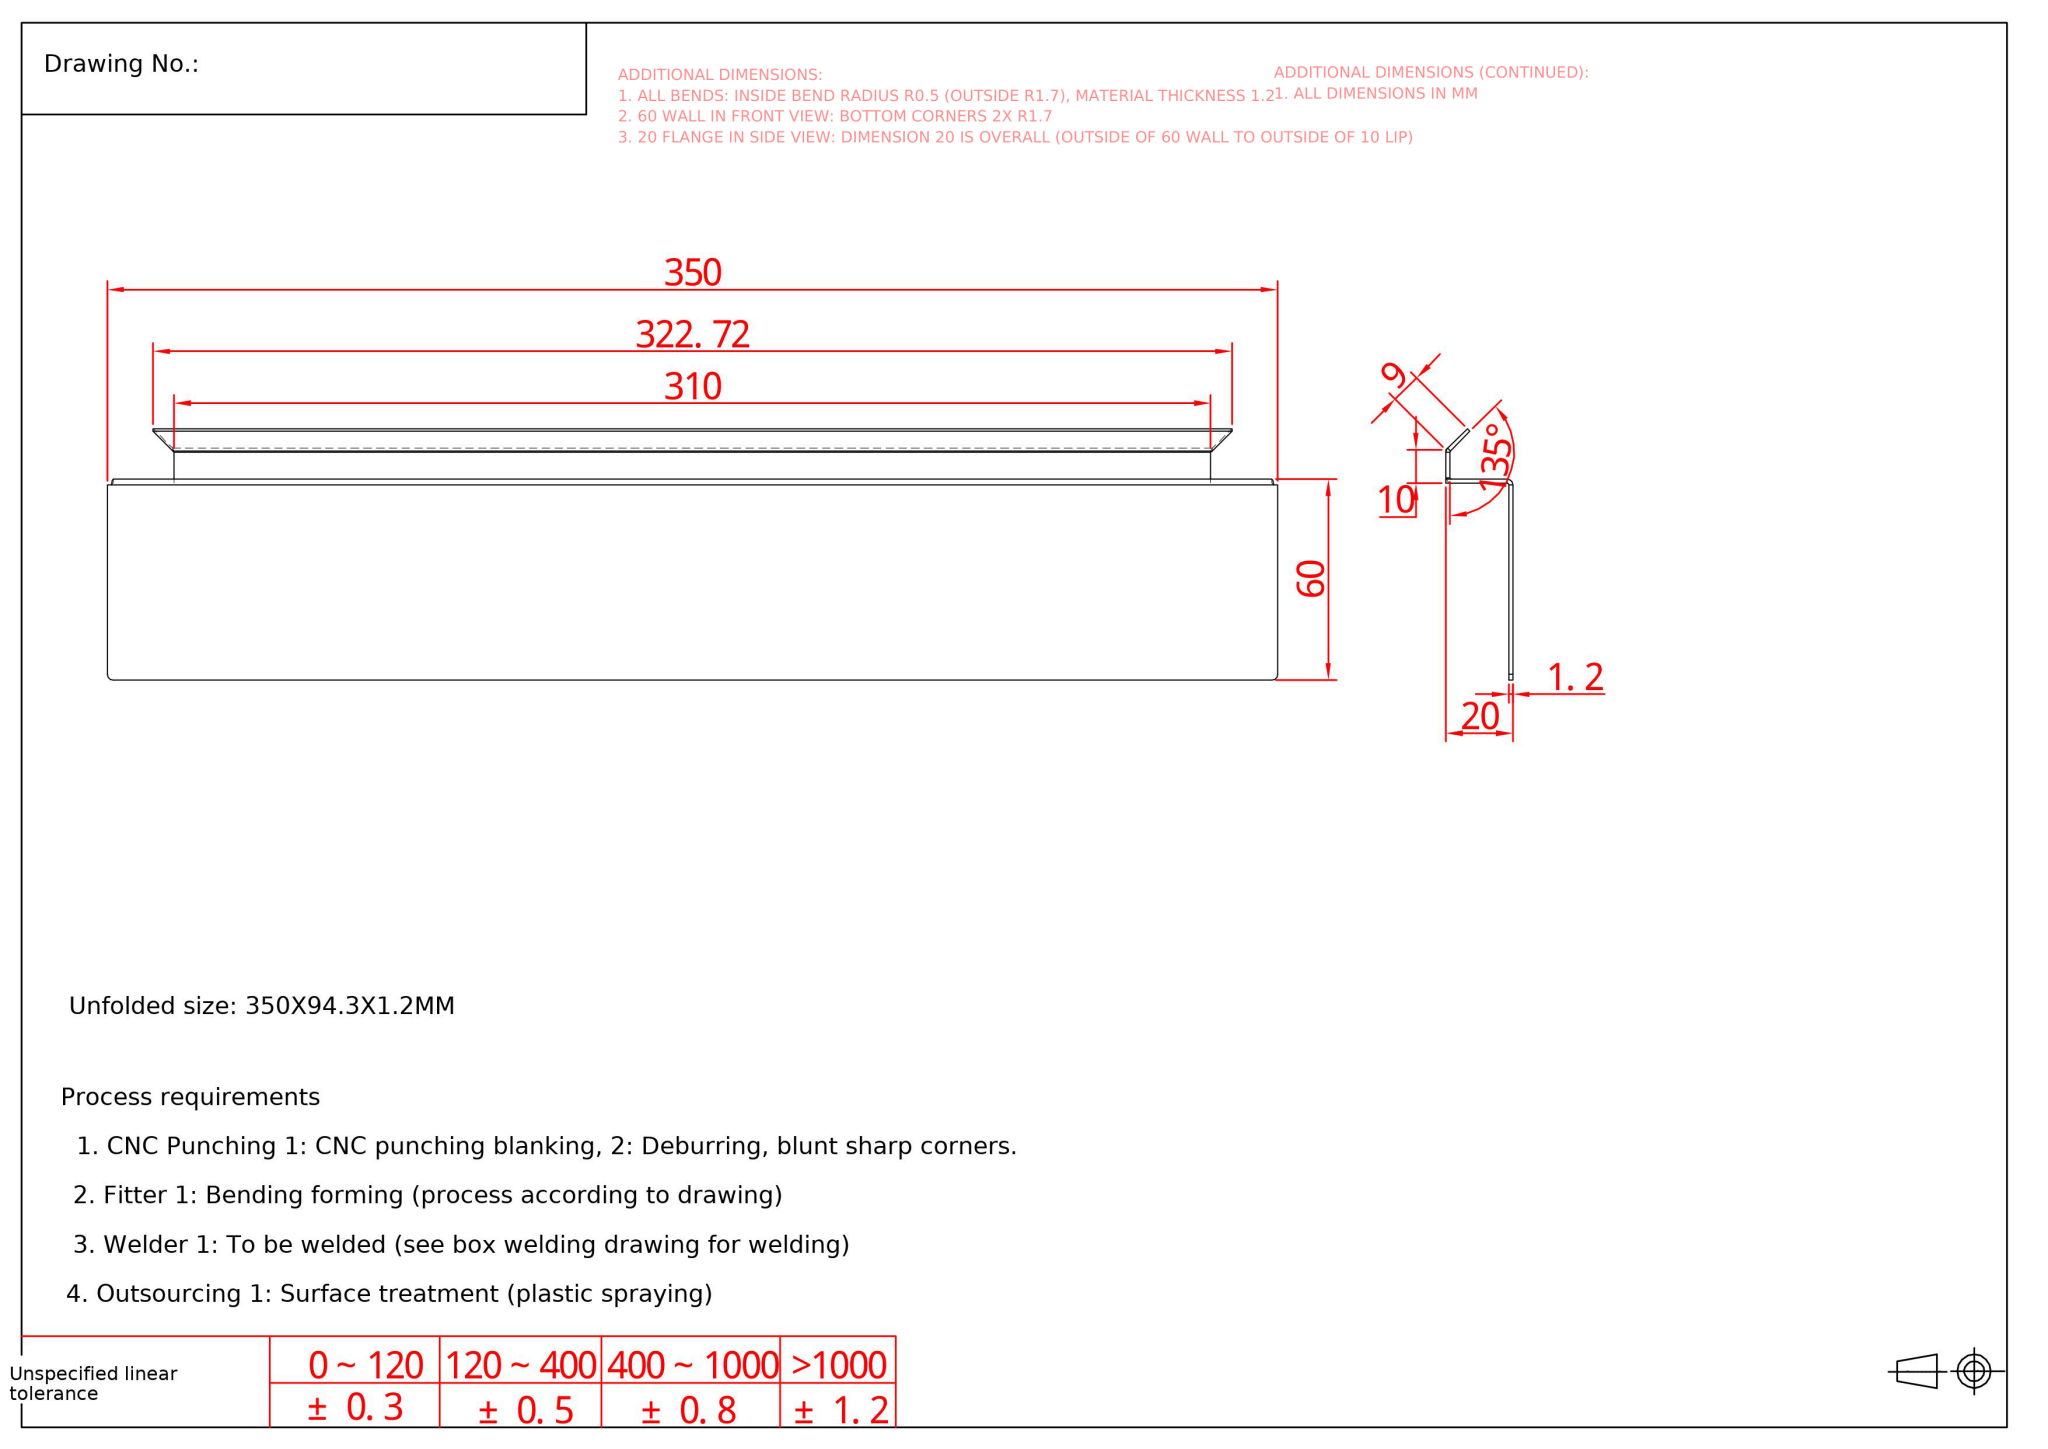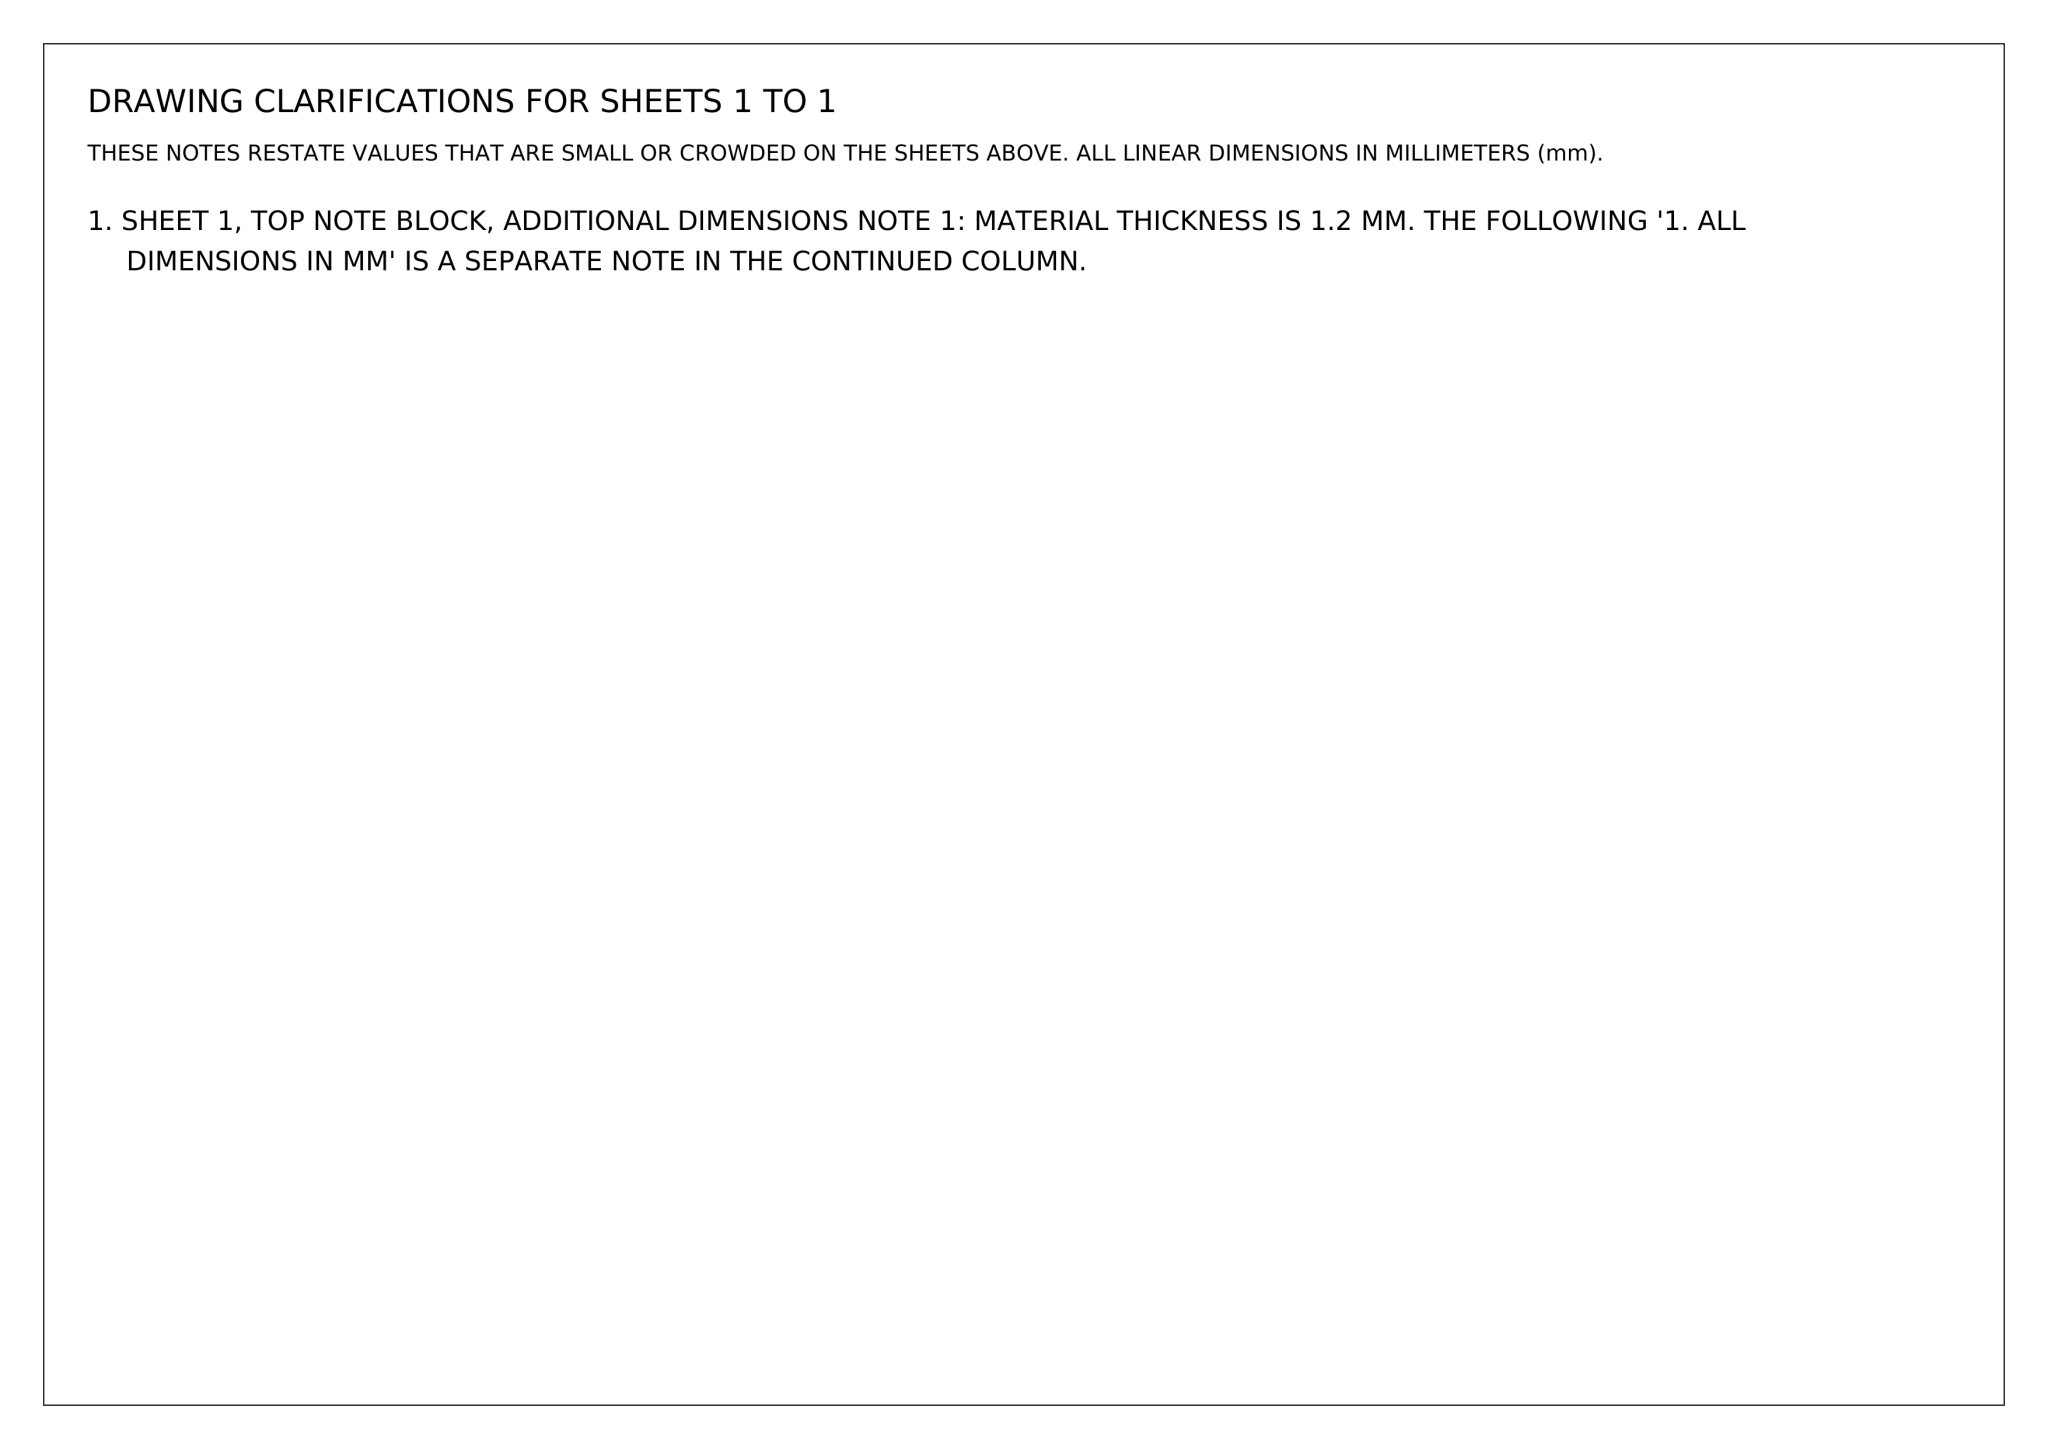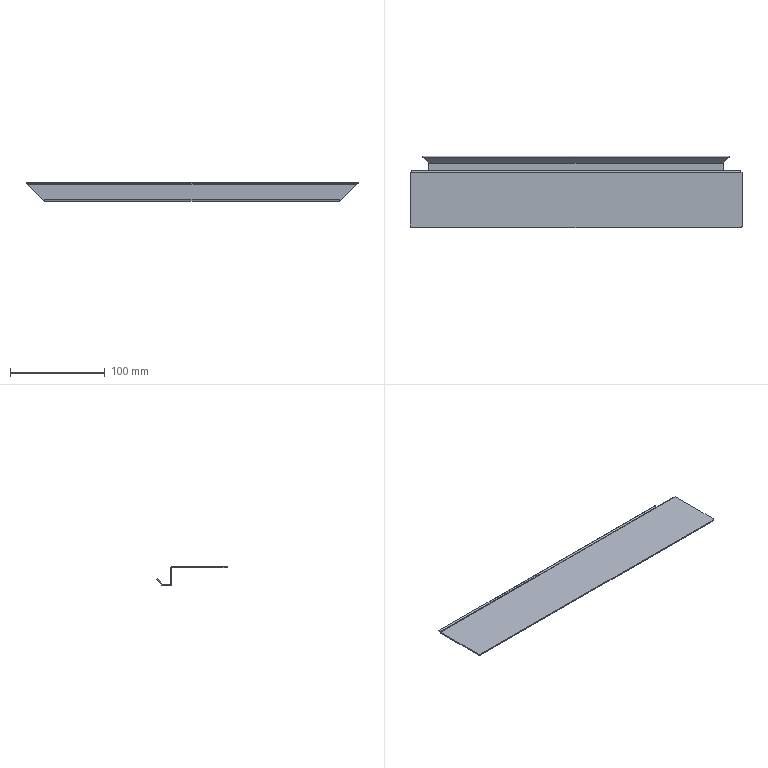Part | NX | mm | 1 solid | 36 faces | box 350 x 75.16 x 20 mm | volume 38725 mm3 | plane 24 | cylinder 8 | spline 4 | commonest cylinder face diameters 3.4 x5 1 x3